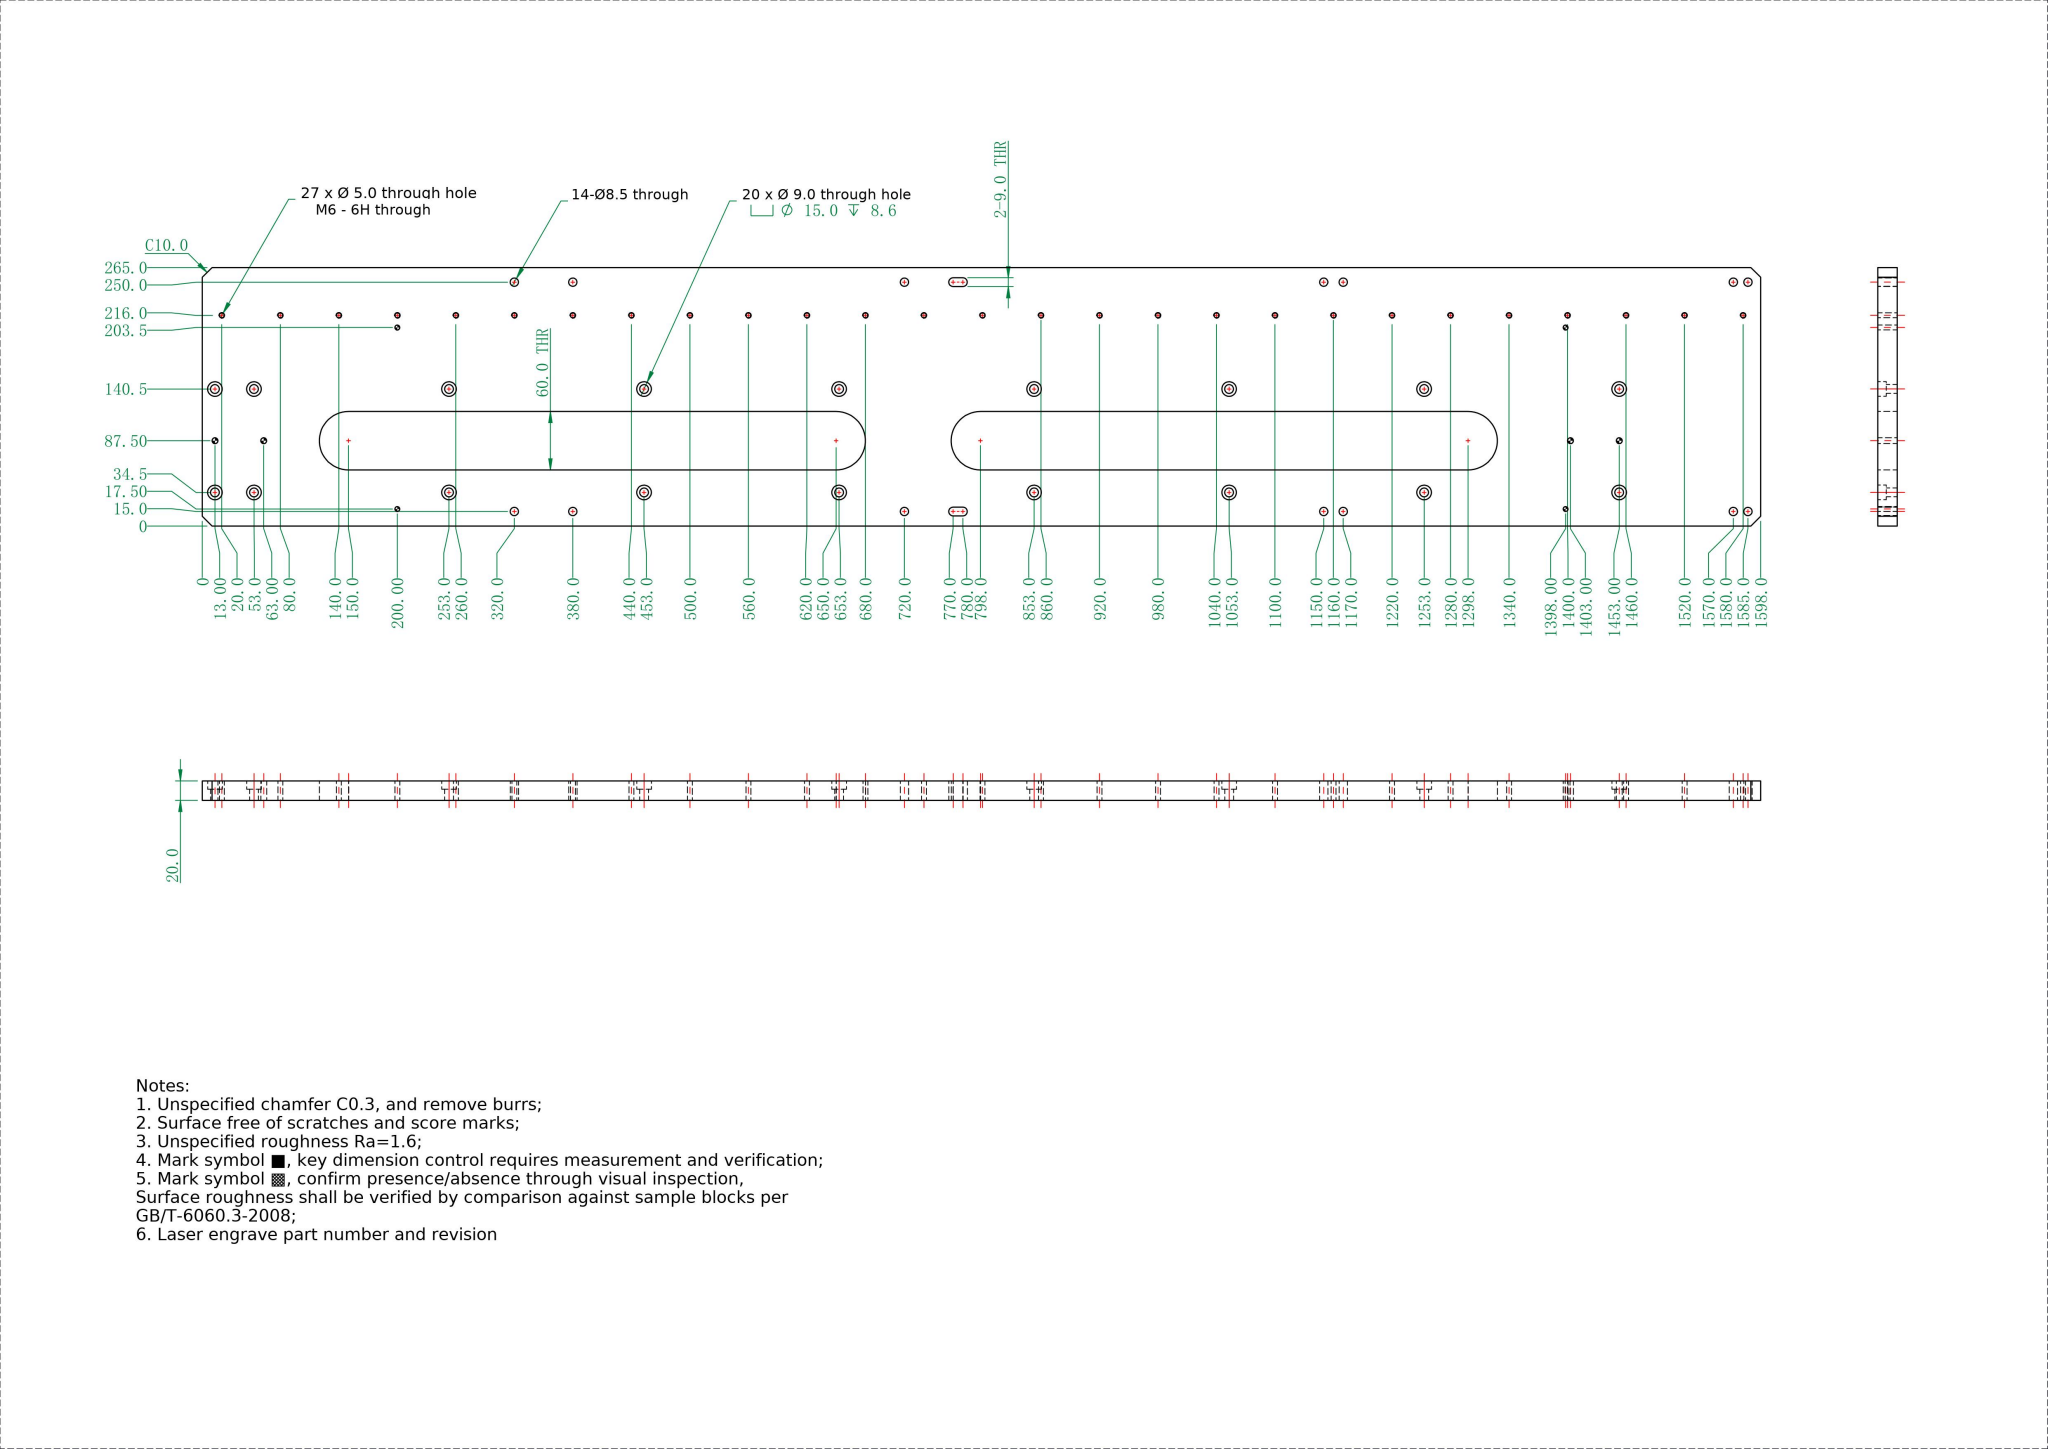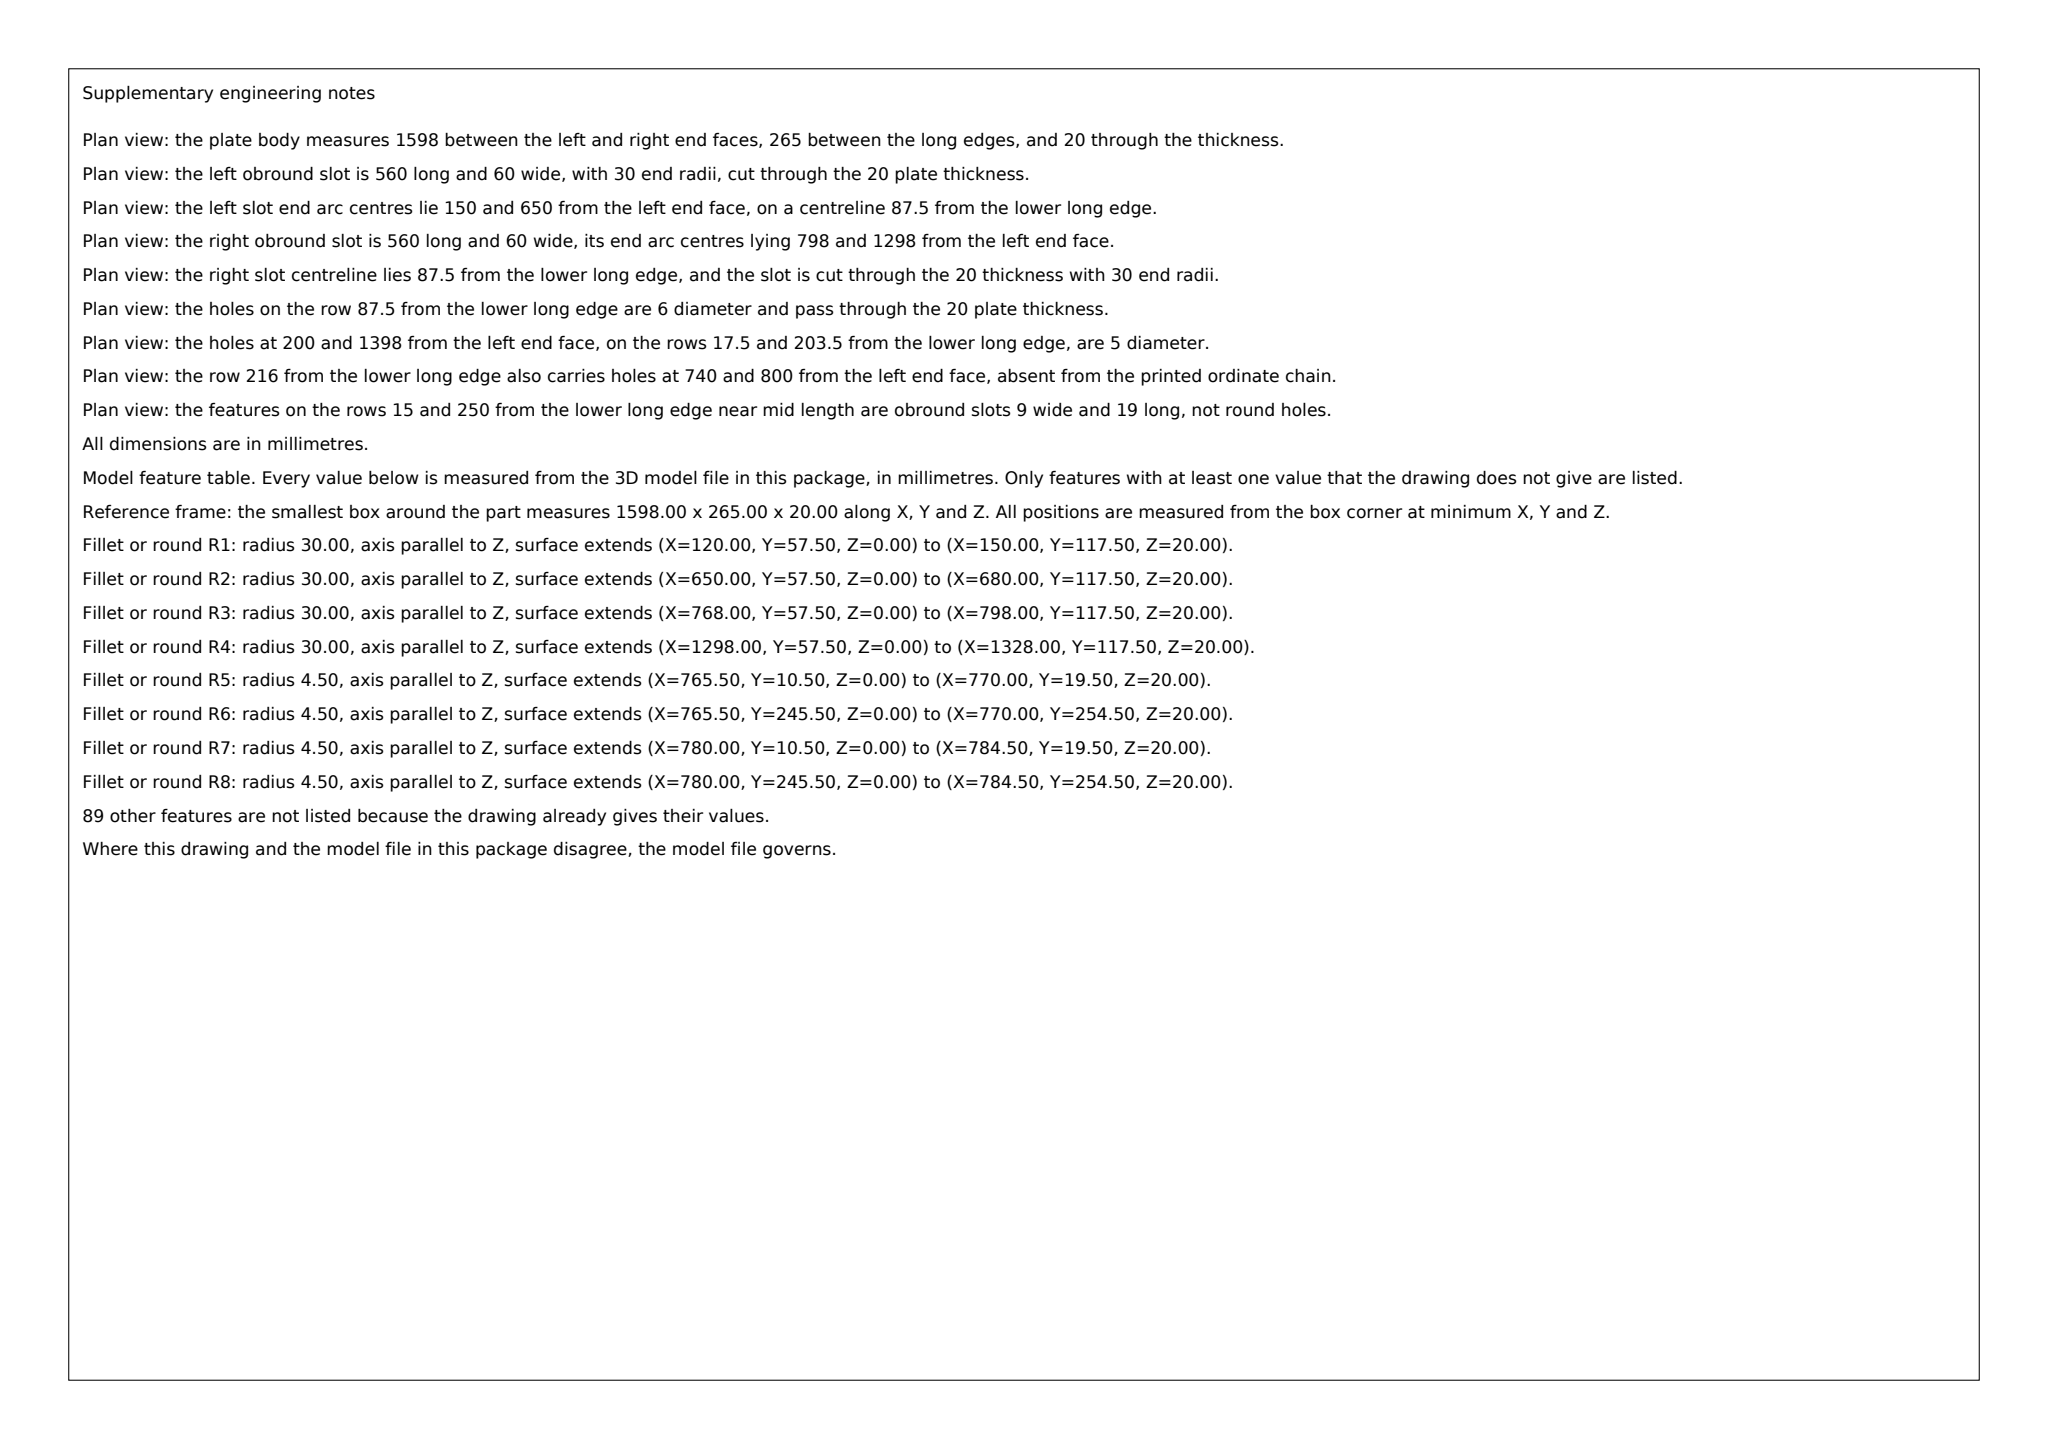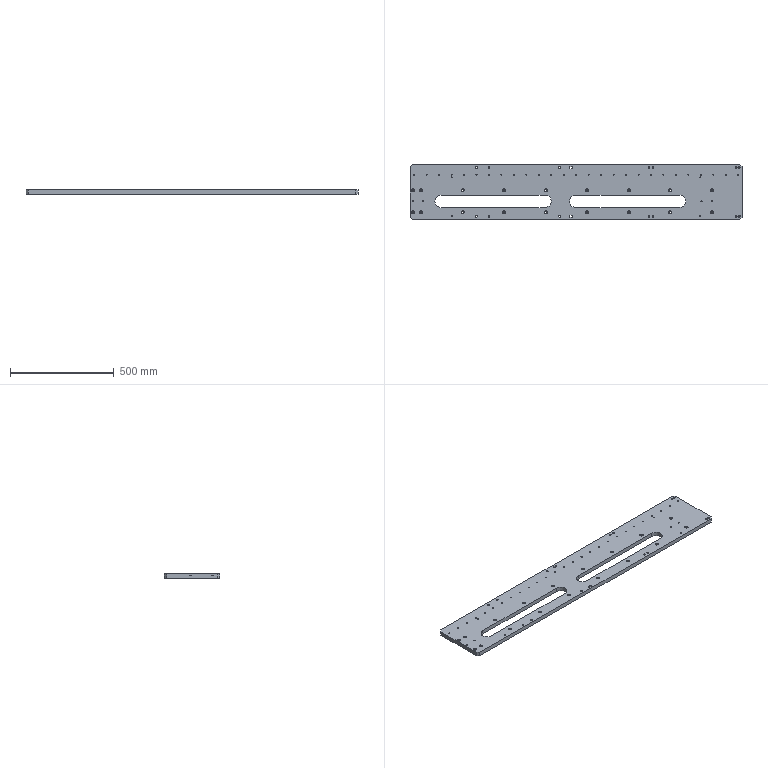Part | SolidWorks | mm | 1 solid | 218 faces | box 1598 x 265 x 20 mm | volume 7075424 mm3 | cylinder 182 | plane 36 | commonest cylinder face diameters 5 x62 9 x42 15 x36 8.5 x28 6 x8 60 x6
Drawing notes:
OVERALL 1598.0 LG x 265.0 W x 20.0 THK | from the solid: bbox_xyz [1598.0,265.0,20.0]; planes x=0/1598, y=0/265, z=0/20
4X C10.0 CORNER CHAMFER, THRU 20.0 THK | from the solid: bbox 1598.0x265.0x20.0; all 4 corners cut 10x10 at 45 deg thru thickness; no fillet radii
2X SLOT 60.0 W, R30.0 ENDS, THRU; CL 87.5 FROM 0 DATUM | from the solid: y-planes 57.5(2) & 117.5(2) => 60.0 W, CL 87.5; full-R ends R30.0; thru 20.0 plate
2X SLOT 9.0 W x 19.0 OAL THRU, CTRS X770.0-780.0, Y15.0 & Y250.0 | from the solid: Ø9.0 z-cyl L20.0 at (770,15),(780,15),(770,250),(780,250) => obround 9.0 W, ctrs 10.0 apart
build123d program:
from build123d import *

# Parameters (mm, degrees)
SKETCH1_W                                       = 1598
SKETCH1_H                                       = 265
BOSS_EXTRUDE1_DEPTH                             = 20
M8_HEX_SOCKET_HEAD_CAP_SCREW_CBORE2_D           = 9
M8_HEX_SOCKET_HEAD_CAP_SCREW_CBORE2_CBORE_D     = 15
M8_HEX_SOCKET_HEAD_CAP_SCREW_CBORE2_CBORE_DEPTH = 8.6
SIZE_MM_DOWEL_PIN_HOLE1_D                       = 6
M6_TAPPED_HOLE1_D                               = 5
SIZE_MM_DOWEL_PIN_HOLE3_D                       = 6
LPATTERN2_COUNT                                 = 27
LPATTERN2_PITCH                                 = 60
SIZE_MM_DOWEL_PIN_HOLE4_D                       = 5
LPATTERN3_COUNT                                 = 2
LPATTERN3_PITCH                                 = 186
SKETCH18_R                                      = 4.25
CUT_EXTRUDE1_DEPTH                              = 1620.947
SKETCH19_R                                      = 4.25
CUT_EXTRUDE2_DEPTH                              = 1620.947
SKETCH21_R                                      = 4.25
CUT_EXTRUDE3_DEPTH                              = 1620.947
CUT_EXTRUDE4_DEPTH                              = 1620.947
CUT_EXTRUDE5_DEPTH                              = 1620.947
CHAMFER1_SIZE                                   = 10


with BuildPart() as part:
    # Sketch1 → Boss-Extrude1 (new body)
    with BuildSketch(Plane.XY):
        with Locations((799, 132.5)):
            Rectangle(SKETCH1_W, SKETCH1_H)
    extrude(amount=BOSS_EXTRUDE1_DEPTH)

    # M8 Hex Socket Head Cap Screw CBORE2 (through all)
    with Locations(Plane.XY.offset(20)):
        with Locations((13, 34.5), (53, 34.5), (53, 140.5), (13, 140.5), (253, 34.5), (253, 140.5), (453, 34.5), (453, 140.5), (653, 34.5), (653, 140.5), (853, 34.5), (853, 140.5), (1053, 34.5), (1053, 140.5), (1253, 34.5), (1253, 140.5), (1453, 34.5), (1453, 140.5), (1653, 34.5), (1653, 140.5)):
            CounterBoreHole(M8_HEX_SOCKET_HEAD_CAP_SCREW_CBORE2_D / 2, M8_HEX_SOCKET_HEAD_CAP_SCREW_CBORE2_CBORE_D / 2, M8_HEX_SOCKET_HEAD_CAP_SCREW_CBORE2_CBORE_DEPTH)

    # Size mm Dowel Pin Hole1 (through all)
    with Locations(Plane.XY.offset(20)):
        with Locations((63, 87.5), (13, 87.5)):
            Hole(SIZE_MM_DOWEL_PIN_HOLE1_D / 2)

    # M6 Tapped Hole1 (through all)
    with Locations(Plane(origin=(0, 0, 0), x_dir=(-1, 0, 0), z_dir=(0, 0, -1))):
        with Locations((-20, 216)):
            m6_tapped_hole1 = Hole(M6_TAPPED_HOLE1_D / 2)

    # Size mm Dowel Pin Hole3 (through all)
    with Locations(Plane.XY.offset(20)):
        with Locations((1453, 87.5), (1403, 87.5)):
            Hole(SIZE_MM_DOWEL_PIN_HOLE3_D / 2)

    # LPattern2: M6 Tapped Hole1 ×27
    with Locations(*[(i * LPATTERN2_PITCH, 0, 0) for i in range(1, LPATTERN2_COUNT)]):
        add(m6_tapped_hole1, mode=Mode.SUBTRACT)

    # Size mm Dowel Pin Hole4 (through all)
    with Locations(Plane(origin=(0, 0, 0), x_dir=(-1, 0, 0), z_dir=(0, 0, -1))):
        with Locations((-1398, 17.5), (-200, 17.5)):
            size_mm_dowel_pin_hole4 = Hole(SIZE_MM_DOWEL_PIN_HOLE4_D / 2)

    # LPattern3: Size mm Dowel Pin Hole4 ×2
    with Locations(*[(0, i * LPATTERN3_PITCH, 0) for i in range(1, LPATTERN3_COUNT)]):
        add(size_mm_dowel_pin_hole4, mode=Mode.SUBTRACT)

    # Sketch18 → Cut-Extrude1 (cut, through all)
    with BuildSketch(Plane(origin=(0, 0, 0), x_dir=(-1, 0, 0), z_dir=(0, 0, -1))):
        with Locations((-380, 250)):
            Circle(SKETCH18_R)
        with Locations((-380, 15)):
            Circle(SKETCH18_R)
        with Locations((-780, 250)):
            Circle(SKETCH18_R)
        with Locations((-780, 15)):
            Circle(SKETCH18_R)
        with Locations((-1150, 250)):
            Circle(SKETCH18_R)
        with Locations((-1150, 15)):
            Circle(SKETCH18_R)
        with Locations((-1585, 15)):
            Circle(SKETCH18_R)
        with Locations((-1585, 250)):
            Circle(SKETCH18_R)
    extrude(amount=-CUT_EXTRUDE1_DEPTH, mode=Mode.SUBTRACT)

    # Sketch19 → Cut-Extrude2 (cut, through all)
    with BuildSketch(Plane(origin=(0, 0, 0), x_dir=(-1, 0, 0), z_dir=(0, 0, -1))):
        with Locations((-320, 15)):
            Circle(SKETCH19_R)
        with Locations((-320, 250)):
            Circle(SKETCH19_R)
        with Locations((-720, 15)):
            Circle(SKETCH19_R)
        with Locations((-720, 250)):
            Circle(SKETCH19_R)
    extrude(amount=-CUT_EXTRUDE2_DEPTH, mode=Mode.SUBTRACT)

    # Sketch21 → Cut-Extrude3 (cut, through all)
    with BuildSketch(Plane(origin=(0, 0, 0), x_dir=(-1, 0, 0), z_dir=(0, 0, -1))):
        with Locations((-1570, 250)):
            Circle(SKETCH21_R)
        with Locations((-1570, 15)):
            Circle(SKETCH21_R)
        with Locations((-1170, 15)):
            Circle(SKETCH21_R)
        with Locations((-1170, 250)):
            Circle(SKETCH21_R)
        with Locations((-770, 15)):
            Circle(SKETCH21_R)
        with Locations((-770, 250)):
            Circle(SKETCH21_R)
    extrude(amount=-CUT_EXTRUDE3_DEPTH, mode=Mode.SUBTRACT)

    # Sketch22 → Cut-Extrude4 (cut, through all)
    with BuildSketch(Plane(origin=(0, 0, 0), x_dir=(-1, 0, 0), z_dir=(0, 0, -1))):
        with BuildLine():
            Line((-780, 19.5), (-770, 19.5))
            ThreePointArc((-770, 19.5), (-765.5, 15), (-770, 10.5))
            Line((-770, 10.5), (-780, 10.5))
            ThreePointArc((-780, 10.5), (-784.5, 15), (-780, 19.5))
        make_face()
        with BuildLine():
            Line((-780, 254.5), (-770, 254.5))
            ThreePointArc((-770, 254.5), (-765.5, 250), (-770, 245.5))
            Line((-770, 245.5), (-780, 245.5))
            ThreePointArc((-780, 245.5), (-784.5, 250), (-780, 254.5))
        make_face()
    extrude(amount=-CUT_EXTRUDE4_DEPTH, mode=Mode.SUBTRACT)

    # Sketch23 → Cut-Extrude5 (cut, through all)
    with BuildSketch(Plane(origin=(0, 0, 0), x_dir=(-1, 0, 0), z_dir=(0, 0, -1))):
        with BuildLine():
            Line((-1298, 117.5), (-798, 117.5))
            ThreePointArc((-798, 117.5), (-768, 87.5), (-798, 57.5))
            Line((-798, 57.5), (-1298, 57.5))
            ThreePointArc((-1298, 57.5), (-1328, 87.5), (-1298, 117.5))
        make_face()
        with BuildLine():
            Line((-650, 117.5), (-150, 117.5))
            ThreePointArc((-150, 117.5), (-120, 87.5), (-150, 57.5))
            Line((-150, 57.5), (-650, 57.5))
            ThreePointArc((-650, 57.5), (-680, 87.5), (-650, 117.5))
        make_face()
    extrude(amount=-CUT_EXTRUDE5_DEPTH, mode=Mode.SUBTRACT)

    # Chamfer1
    chamfer1_edges = [part.edges().sort_by_distance(p)[0] for p in [
        (0, 265, 10),
        (1598, 265, 10),
        (1598, 0, 10),
        (0, 0, 10),
    ]]
    chamfer(chamfer1_edges, length=CHAMFER1_SIZE)


solid = part.part